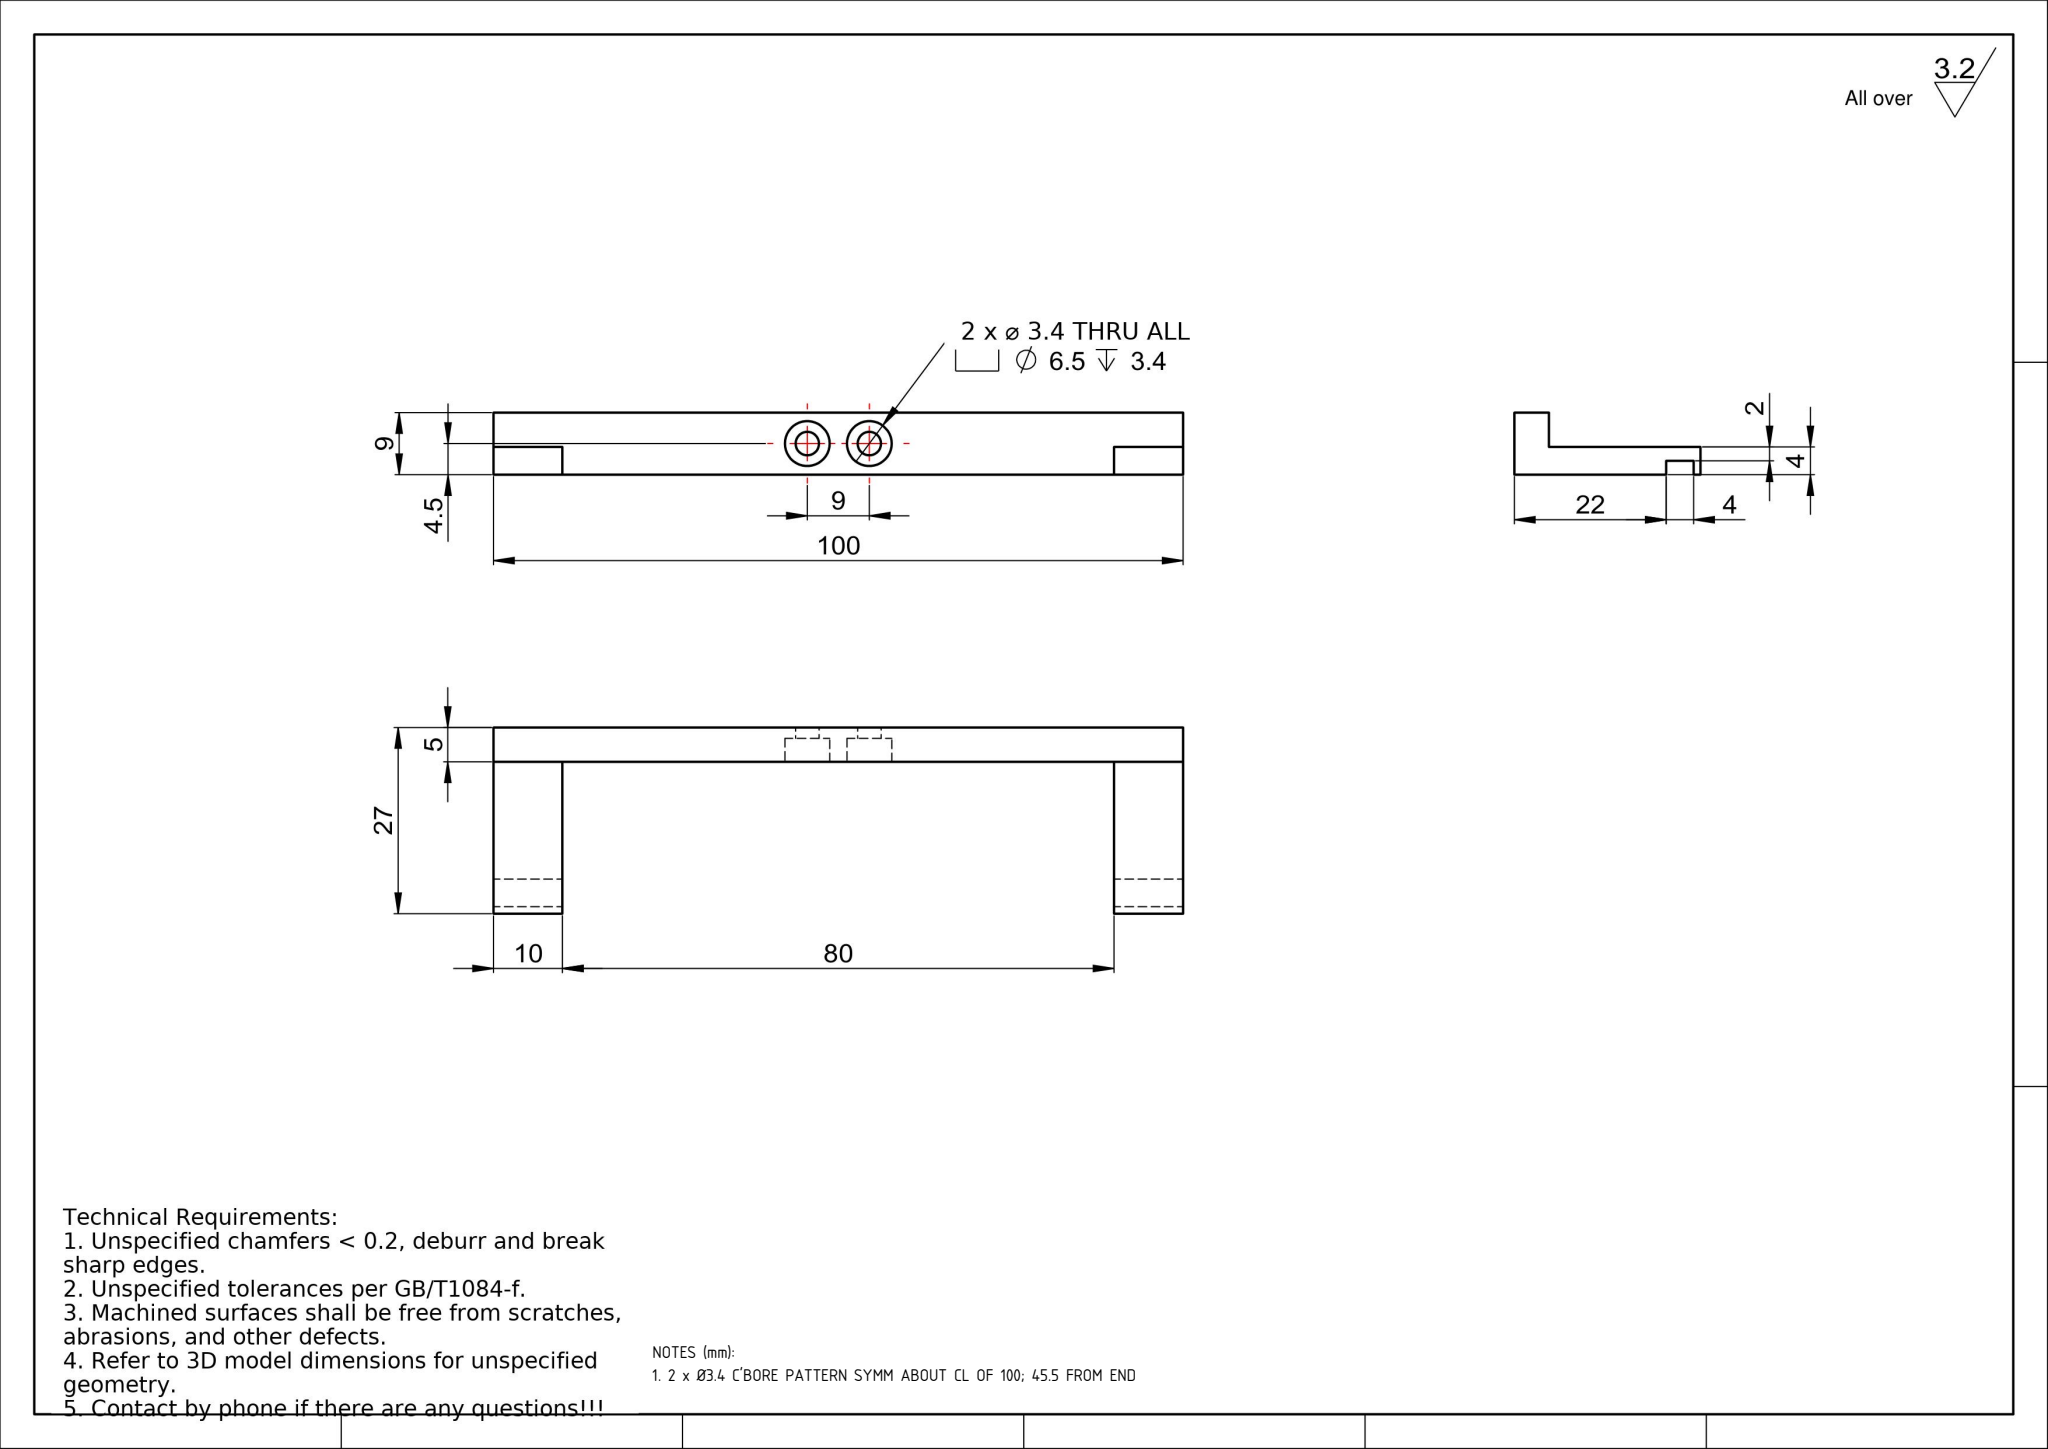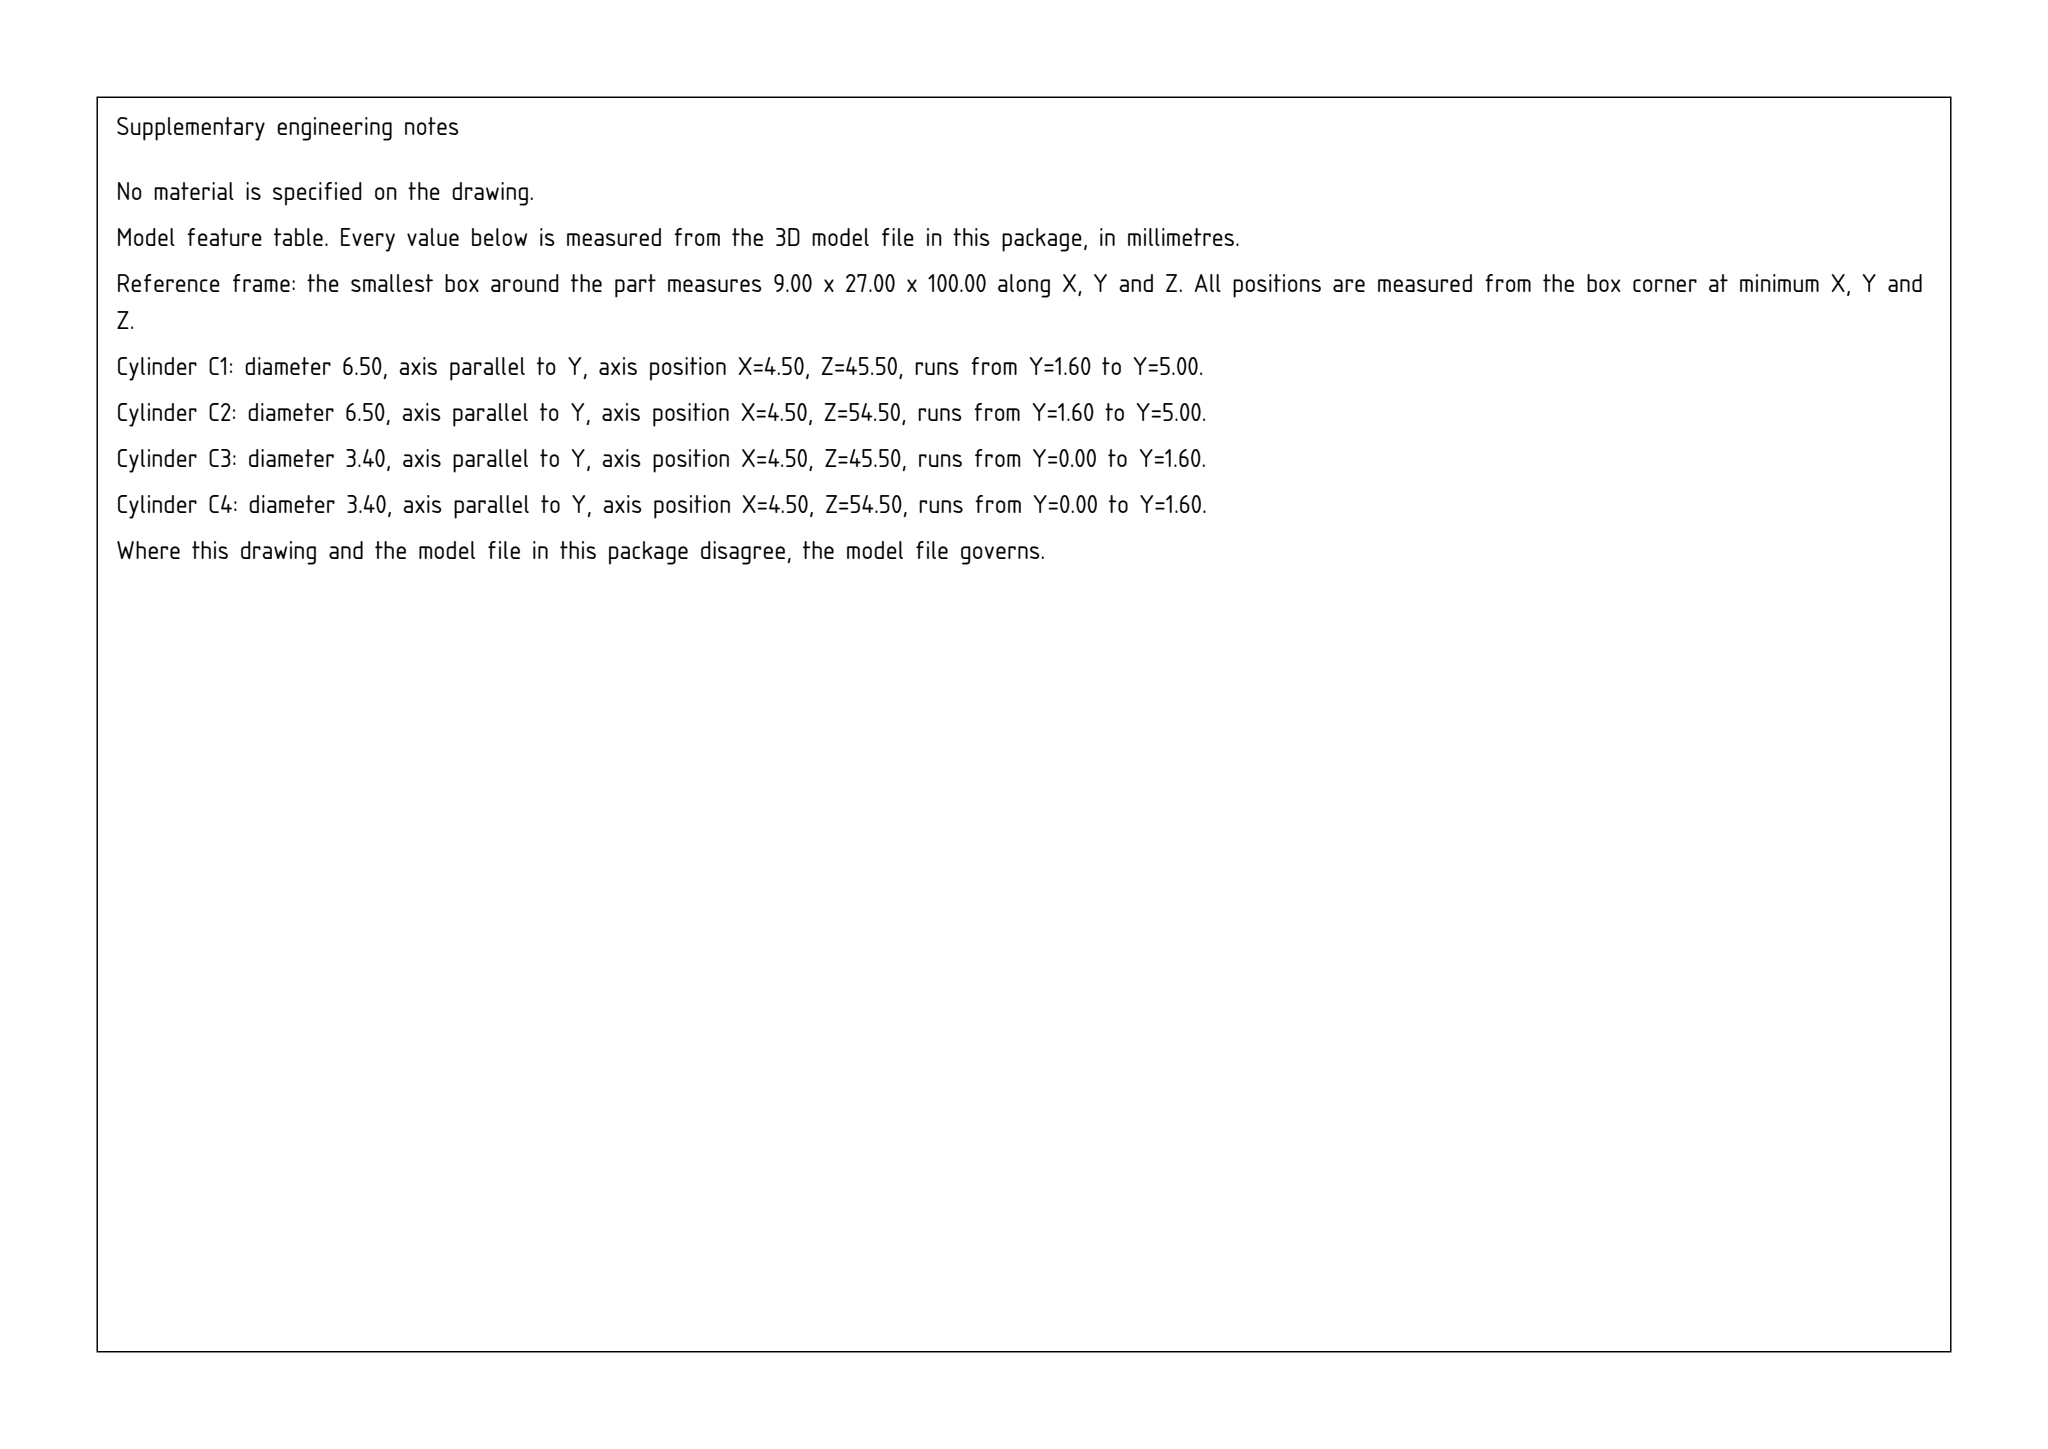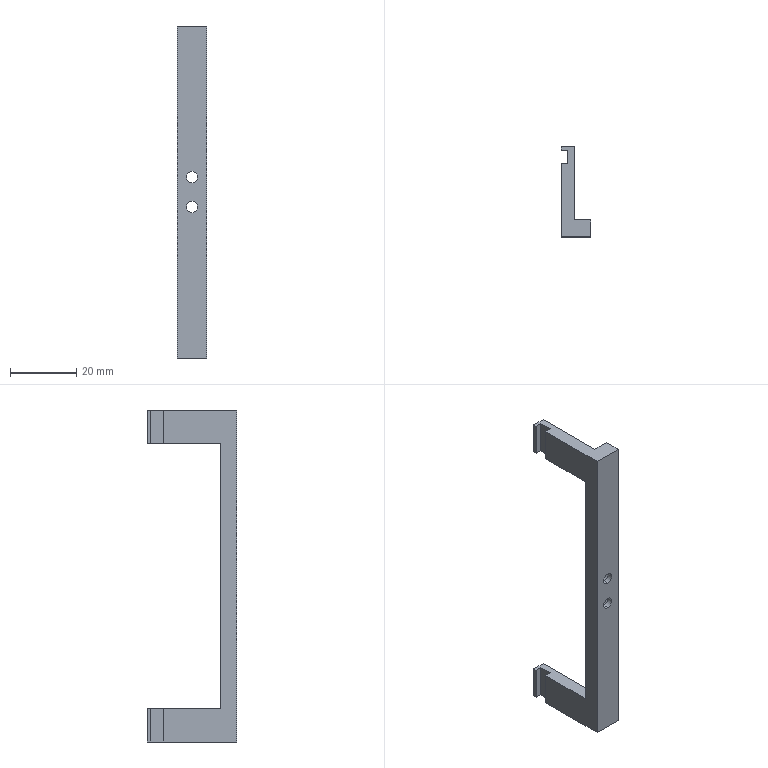Part | SolidWorks | mm | 1 solid | 30 faces | box 9 x 27 x 100 mm | volume 5845 mm3 | plane 22 | cylinder 8 | commonest cylinder face diameters 6.5 x4 3.4 x4
Drawing notes:
2 x Ø3.4 C'BORE PATTERN SYMM ABOUT CL OF 100; 45.5 FROM END | from the solid: Ø3.4/Ø6.5 axes at z=45.5 and 54.5 of 100 length (symmetric about z=50), 9 apart
build123d program:
from build123d import *

# Parameters (mm, degrees)
BOSS_EXTRUDE1_DEPTH                             = 50
SKETCH2_W                                       = 80
SKETCH2_H                                       = 22
CUT_EXTRUDE1_DEPTH                              = 58.044
SKETCH3_W                                       = 2
SKETCH3_H                                       = 4
CUT_EXTRUDE2_DEPTH                              = 104.971
M3_HEX_SOCKET_HEAD_CAP_SCREW_CBORE1_D           = 3.4
M3_HEX_SOCKET_HEAD_CAP_SCREW_CBORE1_CBORE_D     = 6.5
M3_HEX_SOCKET_HEAD_CAP_SCREW_CBORE1_CBORE_DEPTH = 3.4


with BuildPart() as part:
    # Sketch1 → Boss-Extrude1 (new, symmetric)
    with BuildSketch(Plane.XY):
        Polygon((0, 0), (0, 27), (4, 27), (4, 5), (9, 5), (9, 0), align=None)
    extrude(amount=BOSS_EXTRUDE1_DEPTH, both=True)

    # Sketch2 → Cut-Extrude1 (cut, through all)
    with BuildSketch(Plane(origin=(4, 0, 0), x_dir=(0, 0, -1), z_dir=(1, 0, 0))):
        with Locations((0, 16)):
            Rectangle(SKETCH2_W, SKETCH2_H)
    extrude(amount=-CUT_EXTRUDE1_DEPTH, mode=Mode.SUBTRACT)

    # Sketch3 → Cut-Extrude2 (cut, through all)
    with BuildSketch(Plane.XY.offset(50)):
        with Locations((1, 24)):
            Rectangle(SKETCH3_W, SKETCH3_H)
    extrude(amount=-CUT_EXTRUDE2_DEPTH, mode=Mode.SUBTRACT)

    # M3 Hex Socket Head Cap Screw CBORE1 (through all)
    with Locations(Plane(origin=(0, 5, 0), x_dir=(1, 0, 0), z_dir=(0, 1, 0))):
        with Locations((4.5, 4.5), (4.5, -4.5)):
            CounterBoreHole(M3_HEX_SOCKET_HEAD_CAP_SCREW_CBORE1_D / 2, M3_HEX_SOCKET_HEAD_CAP_SCREW_CBORE1_CBORE_D / 2, M3_HEX_SOCKET_HEAD_CAP_SCREW_CBORE1_CBORE_DEPTH)


solid = part.part
STEP:
#1=CARTESIAN_POINT('',(4.5,1.6,-7.75));
#2=VERTEX_POINT('',#1);
#3=CARTESIAN_POINT('',(4.5,1.6,-1.25));
#4=VERTEX_POINT('',#3);
#5=CARTESIAN_POINT('',(4.5,1.6,-4.5));
#6=DIRECTION('',(0.,1.,0.));
#7=DIRECTION('',(0.,0.,1.));
#8=AXIS2_PLACEMENT_3D('',#5,#6,#7);
#9=CIRCLE('',#8,3.25);
#10=EDGE_CURVE('',#2,#4,#9,.T.);
#11=ORIENTED_EDGE('',*,*,#10,.F.);
#12=CARTESIAN_POINT('',(4.5,5.,-7.75));
#13=VERTEX_POINT('',#12);
#14=CARTESIAN_POINT('',(4.5,5.,-7.75));
#15=DIRECTION('',(0.,1.,0.));
#16=VECTOR('',#15,1000.);
#17=LINE('',#14,#16);
#18=EDGE_CURVE('',#2,#13,#17,.T.);
#19=ORIENTED_EDGE('',*,*,#18,.T.);
#20=CARTESIAN_POINT('',(4.5,5.,-1.25));
#21=VERTEX_POINT('',#20);
#22=CARTESIAN_POINT('',(4.5,5.,-4.5));
#23=DIRECTION('',(0.,1.,0.));
#24=DIRECTION('',(0.,0.,1.));
#25=AXIS2_PLACEMENT_3D('',#22,#23,#24);
#26=CIRCLE('',#25,3.25);
#27=EDGE_CURVE('',#13,#21,#26,.T.);
#28=ORIENTED_EDGE('',*,*,#27,.T.);
#29=CARTESIAN_POINT('',(4.5,5.,-1.25));
#30=DIRECTION('',(0.,1.,0.));
#31=VECTOR('',#30,1000.);
#32=LINE('',#29,#31);
#33=EDGE_CURVE('',#4,#21,#32,.T.);
#34=ORIENTED_EDGE('',*,*,#33,.F.);
#35=EDGE_LOOP('',(#11,#19,#28,#34));
#36=FACE_OUTER_BOUND('',#35,.T.);
#37=CARTESIAN_POINT('',(4.5,5.,-4.5));
#38=DIRECTION('',(0.,1.,0.));
#39=DIRECTION('',(0.,0.,1.));
#40=AXIS2_PLACEMENT_3D('',#37,#38,#39);
#41=CYLINDRICAL_SURFACE('',#40,3.25);
#42=ADVANCED_FACE('',(#36),#41,.F.);
#43=CARTESIAN_POINT('',(4.5,-0.,-6.2));
#44=VERTEX_POINT('',#43);
#45=CARTESIAN_POINT('',(4.5,-0.,-2.8));
#46=VERTEX_POINT('',#45);
#47=CARTESIAN_POINT('',(4.5,-0.,-4.5));
#48=DIRECTION('',(0.,1.,0.));
#49=DIRECTION('',(0.,0.,1.));
#50=AXIS2_PLACEMENT_3D('',#47,#48,#49);
#51=CIRCLE('',#50,1.7);
#52=EDGE_CURVE('',#44,#46,#51,.T.);
#53=ORIENTED_EDGE('',*,*,#52,.F.);
#54=CARTESIAN_POINT('',(4.5,1.6,-6.2));
#55=VERTEX_POINT('',#54);
#56=CARTESIAN_POINT('',(4.5,5.,-6.2));
#57=DIRECTION('',(0.,1.,0.));
#58=VECTOR('',#57,1000.);
#59=LINE('',#56,#58);
#60=EDGE_CURVE('',#44,#55,#59,.T.);
#61=ORIENTED_EDGE('',*,*,#60,.T.);
#62=CARTESIAN_POINT('',(4.5,1.6,-2.8));
#63=VERTEX_POINT('',#62);
#64=CARTESIAN_POINT('',(4.5,1.6,-4.5));
#65=DIRECTION('',(0.,1.,0.));
#66=DIRECTION('',(0.,0.,1.));
#67=AXIS2_PLACEMENT_3D('',#64,#65,#66);
#68=CIRCLE('',#67,1.7);
#69=EDGE_CURVE('',#55,#63,#68,.T.);
#70=ORIENTED_EDGE('',*,*,#69,.T.);
#71=CARTESIAN_POINT('',(4.5,5.,-2.8));
#72=DIRECTION('',(0.,1.,0.));
#73=VECTOR('',#72,1000.);
#74=LINE('',#71,#73);
#75=EDGE_CURVE('',#46,#63,#74,.T.);
#76=ORIENTED_EDGE('',*,*,#75,.F.);
#77=EDGE_LOOP('',(#53,#61,#70,#76));
#78=FACE_OUTER_BOUND('',#77,.T.);
#79=CARTESIAN_POINT('',(4.5,5.,-4.5));
#80=DIRECTION('',(0.,1.,0.));
#81=DIRECTION('',(0.,0.,1.));
#82=AXIS2_PLACEMENT_3D('',#79,#80,#81);
#83=CYLINDRICAL_SURFACE('',#82,1.7);
#84=ADVANCED_FACE('',(#78),#83,.F.);
#85=CARTESIAN_POINT('',(4.5,1.6,1.25));
#86=VERTEX_POINT('',#85);
#87=CARTESIAN_POINT('',(4.5,1.6,7.75));
#88=VERTEX_POINT('',#87);
#89=CARTESIAN_POINT('',(4.5,1.6,4.5));
#90=DIRECTION('',(0.,1.,0.));
#91=DIRECTION('',(0.,0.,1.));
#92=AXIS2_PLACEMENT_3D('',#89,#90,#91);
#93=CIRCLE('',#92,3.25);
#94=EDGE_CURVE('',#86,#88,#93,.T.);
#95=ORIENTED_EDGE('',*,*,#94,.F.);
#96=CARTESIAN_POINT('',(4.5,5.,1.25));
#97=VERTEX_POINT('',#96);
#98=CARTESIAN_POINT('',(4.5,5.,1.25));
#99=DIRECTION('',(0.,1.,0.));
#100=VECTOR('',#99,1000.);
#101=LINE('',#98,#100);
#102=EDGE_CURVE('',#86,#97,#101,.T.);
#103=ORIENTED_EDGE('',*,*,#102,.T.);
#104=CARTESIAN_POINT('',(4.5,5.,7.75));
#105=VERTEX_POINT('',#104);
#106=CARTESIAN_POINT('',(4.5,5.,4.5));
#107=DIRECTION('',(0.,1.,0.));
#108=DIRECTION('',(0.,0.,1.));
#109=AXIS2_PLACEMENT_3D('',#106,#107,#108);
#110=CIRCLE('',#109,3.25);
#111=EDGE_CURVE('',#97,#105,#110,.T.);
#112=ORIENTED_EDGE('',*,*,#111,.T.);
#113=CARTESIAN_POINT('',(4.5,5.,7.75));
#114=DIRECTION('',(0.,1.,0.));
#115=VECTOR('',#114,1000.);
#116=LINE('',#113,#115);
#117=EDGE_CURVE('',#88,#105,#116,.T.);
#118=ORIENTED_EDGE('',*,*,#117,.F.);
#119=EDGE_LOOP('',(#95,#103,#112,#118));
#120=FACE_OUTER_BOUND('',#119,.T.);
#121=CARTESIAN_POINT('',(4.5,5.,4.5));
#122=DIRECTION('',(0.,1.,0.));
#123=DIRECTION('',(0.,0.,1.));
#124=AXIS2_PLACEMENT_3D('',#121,#122,#123);
#125=CYLINDRICAL_SURFACE('',#124,3.25);
#126=ADVANCED_FACE('',(#120),#125,.F.);
#127=CARTESIAN_POINT('',(4.5,-0.,2.8));
#128=VERTEX_POINT('',#127);
#129=CARTESIAN_POINT('',(4.5,-0.,6.2));
#130=VERTEX_POINT('',#129);
#131=CARTESIAN_POINT('',(4.5,-0.,4.5));
#132=DIRECTION('',(0.,1.,0.));
#133=DIRECTION('',(0.,0.,1.));
#134=AXIS2_PLACEMENT_3D('',#131,#132,#133);
#135=CIRCLE('',#134,1.7);
#136=EDGE_CURVE('',#128,#130,#135,.T.);
#137=ORIENTED_EDGE('',*,*,#136,.F.);
#138=CARTESIAN_POINT('',(4.5,1.6,2.8));
#139=VERTEX_POINT('',#138);
#140=CARTESIAN_POINT('',(4.5,5.,2.8));
#141=DIRECTION('',(0.,1.,0.));
#142=VECTOR('',#141,1000.);
#143=LINE('',#140,#142);
#144=EDGE_CURVE('',#128,#139,#143,.T.);
#145=ORIENTED_EDGE('',*,*,#144,.T.);
#146=CARTESIAN_POINT('',(4.5,1.6,6.2));
#147=VERTEX_POINT('',#146);
#148=CARTESIAN_POINT('',(4.5,1.6,4.5));
#149=DIRECTION('',(0.,1.,0.));
#150=DIRECTION('',(0.,0.,1.));
#151=AXIS2_PLACEMENT_3D('',#148,#149,#150);
#152=CIRCLE('',#151,1.7);
#153=EDGE_CURVE('',#139,#147,#152,.T.);
#154=ORIENTED_EDGE('',*,*,#153,.T.);
#155=CARTESIAN_POINT('',(4.5,5.,6.2));
#156=DIRECTION('',(0.,1.,0.));
#157=VECTOR('',#156,1000.);
#158=LINE('',#155,#157);
#159=EDGE_CURVE('',#130,#147,#158,.T.);
#160=ORIENTED_EDGE('',*,*,#159,.F.);
#161=EDGE_LOOP('',(#137,#145,#154,#160));
#162=FACE_OUTER_BOUND('',#161,.T.);
#163=CARTESIAN_POINT('',(4.5,5.,4.5));
#164=DIRECTION('',(0.,1.,0.));
#165=DIRECTION('',(0.,0.,1.));
#166=AXIS2_PLACEMENT_3D('',#163,#164,#165);
#167=CYLINDRICAL_SURFACE('',#166,1.7);
#168=ADVANCED_FACE('',(#162),#167,.F.);
#169=CARTESIAN_POINT('',(-0.,27.,40.));
#170=VERTEX_POINT('',#169);
#171=CARTESIAN_POINT('',(0.,26.,40.));
#172=VERTEX_POINT('',#171);
#173=CARTESIAN_POINT('',(-0.,27.,40.));
#174=DIRECTION('',(0.,-1.,0.));
#175=VECTOR('',#174,1000.);
#176=LINE('',#173,#175);
#177=EDGE_CURVE('',#170,#172,#176,.T.);
#178=ORIENTED_EDGE('',*,*,#177,.T.);
#179=CARTESIAN_POINT('',(0.,26.,50.));
#180=VERTEX_POINT('',#179);
#181=CARTESIAN_POINT('',(0.,26.,-50.));
#182=DIRECTION('',(0.,0.,1.));
#183=VECTOR('',#182,1000.);
#184=LINE('',#181,#183);
#185=EDGE_CURVE('',#172,#180,#184,.T.);
#186=ORIENTED_EDGE('',*,*,#185,.T.);
#187=CARTESIAN_POINT('',(0.,27.,50.));
#188=VERTEX_POINT('',#187);
#189=CARTESIAN_POINT('',(0.,0.,50.));
#190=DIRECTION('',(0.,-1.,0.));
#191=VECTOR('',#190,1000.);
#192=LINE('',#189,#191);
#193=EDGE_CURVE('',#188,#180,#192,.T.);
#194=ORIENTED_EDGE('',*,*,#193,.F.);
#195=CARTESIAN_POINT('',(0.,27.,50.));
#196=DIRECTION('',(0.,0.,-1.));
#197=VECTOR('',#196,1000.);
#198=LINE('',#195,#197);
#199=EDGE_CURVE('',#188,#170,#198,.T.);
#200=ORIENTED_EDGE('',*,*,#199,.T.);
#201=EDGE_LOOP('',(#178,#186,#194,#200));
#202=FACE_OUTER_BOUND('',#201,.T.);
#203=CARTESIAN_POINT('',(0.,0.,50.));
#204=DIRECTION('',(1.,0.,0.));
#205=DIRECTION('',(0.,0.,-1.));
#206=AXIS2_PLACEMENT_3D('',#203,#204,#205);
#207=PLANE('',#206);
#208=ADVANCED_FACE('',(#202),#207,.F.);
#209=CARTESIAN_POINT('',(0.,27.,-50.));
#210=VERTEX_POINT('',#209);
#211=CARTESIAN_POINT('',(0.,26.,-50.));
#212=VERTEX_POINT('',#211);
#213=CARTESIAN_POINT('',(0.,0.,-50.));
#214=DIRECTION('',(0.,-1.,0.));
#215=VECTOR('',#214,1000.);
#216=LINE('',#213,#215);
#217=EDGE_CURVE('',#210,#212,#216,.T.);
#218=ORIENTED_EDGE('',*,*,#217,.T.);
#219=CARTESIAN_POINT('',(0.,26.,-40.));
#220=VERTEX_POINT('',#219);
#221=CARTESIAN_POINT('',(0.,26.,-50.));
#222=DIRECTION('',(0.,0.,1.));
#223=VECTOR('',#222,1000.);
#224=LINE('',#221,#223);
#225=EDGE_CURVE('',#212,#220,#224,.T.);
#226=ORIENTED_EDGE('',*,*,#225,.T.);
#227=CARTESIAN_POINT('',(-0.,27.,-40.));
#228=VERTEX_POINT('',#227);
#229=CARTESIAN_POINT('',(-0.,27.,-40.));
#230=DIRECTION('',(-0.,1.,0.));
#231=VECTOR('',#230,1000.);
#232=LINE('',#229,#231);
#233=EDGE_CURVE('',#220,#228,#232,.T.);
#234=ORIENTED_EDGE('',*,*,#233,.T.);
#235=CARTESIAN_POINT('',(0.,27.,50.));
#236=DIRECTION('',(0.,0.,-1.));
#237=VECTOR('',#236,1000.);
#238=LINE('',#235,#237);
#239=EDGE_CURVE('',#228,#210,#238,.T.);
#240=ORIENTED_EDGE('',*,*,#239,.T.);
#241=EDGE_LOOP('',(#218,#226,#234,#240));
#242=FACE_OUTER_BOUND('',#241,.T.);
#243=CARTESIAN_POINT('',(0.,0.,50.));
#244=DIRECTION('',(1.,0.,0.));
#245=DIRECTION('',(0.,0.,-1.));
#246=AXIS2_PLACEMENT_3D('',#243,#244,#245);
#247=PLANE('',#246);
#248=ADVANCED_FACE('',(#242),#247,.F.);
#249=CARTESIAN_POINT('',(4.,5.,50.));
#250=VERTEX_POINT('',#249);
#251=CARTESIAN_POINT('',(4.,5.,40.));
#252=VERTEX_POINT('',#251);
#253=CARTESIAN_POINT('',(4.,5.,50.));
#254=DIRECTION('',(0.,0.,-1.));
#255=VECTOR('',#254,1000.);
#256=LINE('',#253,#255);
#257=EDGE_CURVE('',#250,#252,#256,.T.);
#258=ORIENTED_EDGE('',*,*,#257,.T.);
#259=CARTESIAN_POINT('',(4.,27.,40.));
#260=VERTEX_POINT('',#259);
#261=CARTESIAN_POINT('',(4.,27.,40.));
#262=DIRECTION('',(0.,-1.,0.));
#263=VECTOR('',#262,1000.);
#264=LINE('',#261,#263);
#265=EDGE_CURVE('',#260,#252,#264,.T.);
#266=ORIENTED_EDGE('',*,*,#265,.F.);
#267=CARTESIAN_POINT('',(4.,27.,50.));
#268=VERTEX_POINT('',#267);
#269=CARTESIAN_POINT('',(4.,27.,50.));
#270=DIRECTION('',(0.,0.,-1.));
#271=VECTOR('',#270,1000.);
#272=LINE('',#269,#271);
#273=EDGE_CURVE('',#268,#260,#272,.T.);
#274=ORIENTED_EDGE('',*,*,#273,.F.);
#275=CARTESIAN_POINT('',(4.,27.,50.));
#276=DIRECTION('',(-0.,1.,0.));
#277=VECTOR('',#276,1000.);
#278=LINE('',#275,#277);
#279=EDGE_CURVE('',#250,#268,#278,.T.);
#280=ORIENTED_EDGE('',*,*,#279,.F.);
#281=EDGE_LOOP('',(#258,#266,#274,#280));
#282=FACE_OUTER_BOUND('',#281,.T.);
#283=CARTESIAN_POINT('',(4.,27.,50.));
#284=DIRECTION('',(-1.,-0.,0.));
#285=DIRECTION('',(0.,-1.,0.));
#286=AXIS2_PLACEMENT_3D('',#283,#284,#285);
#287=PLANE('',#286);
#288=ADVANCED_FACE('',(#282),#287,.F.);
#289=ORIENTED_EDGE('',*,*,#273,.T.);
#290=CARTESIAN_POINT('',(-0.,27.,40.));
#291=DIRECTION('',(1.,0.,0.));
#292=VECTOR('',#291,1000.);
#293=LINE('',#290,#292);
#294=EDGE_CURVE('',#170,#260,#293,.T.);
#295=ORIENTED_EDGE('',*,*,#294,.F.);
#296=ORIENTED_EDGE('',*,*,#199,.F.);
#297=CARTESIAN_POINT('',(0.,27.,50.));
#298=DIRECTION('',(-1.,0.,0.));
#299=VECTOR('',#298,1000.);
#300=LINE('',#297,#299);
#301=EDGE_CURVE('',#268,#188,#300,.T.);
#302=ORIENTED_EDGE('',*,*,#301,.F.);
#303=EDGE_LOOP('',(#289,#295,#296,#302));
#304=FACE_OUTER_BOUND('',#303,.T.);
#305=CARTESIAN_POINT('',(0.,27.,50.));
#306=DIRECTION('',(0.,-1.,0.));
#307=DIRECTION('',(0.,0.,-1.));
#308=AXIS2_PLACEMENT_3D('',#305,#306,#307);
#309=PLANE('',#308);
#310=ADVANCED_FACE('',(#304),#309,.F.);
#311=CARTESIAN_POINT('',(4.5,-0.,-4.5));
#312=DIRECTION('',(0.,1.,0.));
#313=DIRECTION('',(0.,0.,1.));
#314=AXIS2_PLACEMENT_3D('',#311,#312,#313);
#315=CIRCLE('',#314,1.7);
#316=EDGE_CURVE('',#46,#44,#315,.T.);
#317=ORIENTED_EDGE('',*,*,#316,.T.);
#318=ORIENTED_EDGE('',*,*,#52,.T.);
#319=EDGE_LOOP('',(#317,#318));
#320=FACE_BOUND('',#319,.T.);
#321=CARTESIAN_POINT('',(4.5,-0.,4.5));
#322=DIRECTION('',(0.,1.,0.));
#323=DIRECTION('',(0.,0.,1.));
#324=AXIS2_PLACEMENT_3D('',#321,#322,#323);
#325=CIRCLE('',#324,1.7);
#326=EDGE_CURVE('',#130,#128,#325,.T.);
#327=ORIENTED_EDGE('',*,*,#326,.T.);
#328=ORIENTED_EDGE('',*,*,#136,.T.);
#329=EDGE_LOOP('',(#327,#328));
#330=FACE_BOUND('',#329,.T.);
#331=CARTESIAN_POINT('',(0.,0.,-50.));
#332=VERTEX_POINT('',#331);
#333=CARTESIAN_POINT('',(9.,-0.,-50.));
#334=VERTEX_POINT('',#333);
#335=CARTESIAN_POINT('',(9.,-0.,-50.));
#336=DIRECTION('',(1.,-0.,0.));
#337=VECTOR('',#336,1000.);
#338=LINE('',#335,#337);
#339=EDGE_CURVE('',#332,#334,#338,.T.);
#340=ORIENTED_EDGE('',*,*,#339,.T.);
#341=CARTESIAN_POINT('',(9.,-0.,50.));
#342=VERTEX_POINT('',#341);
#343=CARTESIAN_POINT('',(9.,-0.,50.));
#344=DIRECTION('',(0.,0.,-1.));
#345=VECTOR('',#344,1000.);
#346=LINE('',#343,#345);
#347=EDGE_CURVE('',#342,#334,#346,.T.);
#348=ORIENTED_EDGE('',*,*,#347,.F.);
#349=CARTESIAN_POINT('',(0.,0.,50.));
#350=VERTEX_POINT('',#349);
#351=CARTESIAN_POINT('',(9.,-0.,50.));
#352=DIRECTION('',(1.,-0.,0.));
#353=VECTOR('',#352,1000.);
#354=LINE('',#351,#353);
#355=EDGE_CURVE('',#350,#342,#354,.T.);
#356=ORIENTED_EDGE('',*,*,#355,.F.);
#357=CARTESIAN_POINT('',(0.,0.,50.));
#358=DIRECTION('',(0.,0.,-1.));
#359=VECTOR('',#358,1000.);
#360=LINE('',#357,#359);
#361=EDGE_CURVE('',#350,#332,#360,.T.);
#362=ORIENTED_EDGE('',*,*,#361,.T.);
#363=EDGE_LOOP('',(#340,#348,#356,#362));
#364=FACE_OUTER_BOUND('',#363,.T.);
#365=CARTESIAN_POINT('',(9.,-0.,50.));
#366=DIRECTION('',(0.,1.,0.));
#367=DIRECTION('',(-1.,0.,0.));
#368=AXIS2_PLACEMENT_3D('',#365,#366,#367);
#369=PLANE('',#368);
#370=ADVANCED_FACE('',(#320,#330,#364),#369,.F.);
#371=CARTESIAN_POINT('',(9.,5.,-50.));
#372=VERTEX_POINT('',#371);
#373=CARTESIAN_POINT('',(9.,5.,-50.));
#374=DIRECTION('',(-0.,1.,0.));
#375=VECTOR('',#374,1000.);
#376=LINE('',#373,#375);
#377=EDGE_CURVE('',#334,#372,#376,.T.);
#378=ORIENTED_EDGE('',*,*,#377,.T.);
#379=CARTESIAN_POINT('',(9.,5.,50.));
#380=VERTEX_POINT('',#379);
#381=CARTESIAN_POINT('',(9.,5.,50.));
#382=DIRECTION('',(0.,0.,-1.));
#383=VECTOR('',#382,1000.);
#384=LINE('',#381,#383);
#385=EDGE_CURVE('',#380,#372,#384,.T.);
#386=ORIENTED_EDGE('',*,*,#385,.F.);
#387=CARTESIAN_POINT('',(9.,5.,50.));
#388=DIRECTION('',(-0.,1.,0.));
#389=VECTOR('',#388,1000.);
#390=LINE('',#387,#389);
#391=EDGE_CURVE('',#342,#380,#390,.T.);
#392=ORIENTED_EDGE('',*,*,#391,.F.);
#393=ORIENTED_EDGE('',*,*,#347,.T.);
#394=EDGE_LOOP('',(#378,#386,#392,#393));
#395=FACE_OUTER_BOUND('',#394,.T.);
#396=CARTESIAN_POINT('',(9.,5.,50.));
#397=DIRECTION('',(-1.,-0.,0.));
#398=DIRECTION('',(0.,-1.,0.));
#399=AXIS2_PLACEMENT_3D('',#396,#397,#398);
#400=PLANE('',#399);
#401=ADVANCED_FACE('',(#395),#400,.F.);
#402=CARTESIAN_POINT('',(4.5,5.,-4.5));
#403=DIRECTION('',(0.,1.,0.));
#404=DIRECTION('',(0.,0.,1.));
#405=AXIS2_PLACEMENT_3D('',#402,#403,#404);
#406=CIRCLE('',#405,3.25);
#407=EDGE_CURVE('',#21,#13,#406,.T.);
#408=ORIENTED_EDGE('',*,*,#407,.F.);
#409=ORIENTED_EDGE('',*,*,#27,.F.);
#410=EDGE_LOOP('',(#408,#409));
#411=FACE_BOUND('',#410,.T.);
#412=CARTESIAN_POINT('',(4.5,5.,4.5));
#413=DIRECTION('',(0.,1.,0.));
#414=DIRECTION('',(0.,0.,1.));
#415=AXIS2_PLACEMENT_3D('',#412,#413,#414);
#416=CIRCLE('',#415,3.25);
#417=EDGE_CURVE('',#105,#97,#416,.T.);
#418=ORIENTED_EDGE('',*,*,#417,.F.);
#419=ORIENTED_EDGE('',*,*,#111,.F.);
#420=EDGE_LOOP('',(#418,#419));
#421=FACE_BOUND('',#420,.T.);
#422=CARTESIAN_POINT('',(4.,5.,-50.));
#423=VERTEX_POINT('',#422);
#424=CARTESIAN_POINT('',(4.,5.,-50.));
#425=DIRECTION('',(-1.,0.,0.));
#426=VECTOR('',#425,1000.);
#427=LINE('',#424,#426);
#428=EDGE_CURVE('',#372,#423,#427,.T.);
#429=ORIENTED_EDGE('',*,*,#428,.T.);
#430=CARTESIAN_POINT('',(4.,5.,-40.));
#431=VERTEX_POINT('',#430);
#432=CARTESIAN_POINT('',(4.,5.,50.));
#433=DIRECTION('',(0.,0.,-1.));
#434=VECTOR('',#433,1000.);
#435=LINE('',#432,#434);
#436=EDGE_CURVE('',#431,#423,#435,.T.);
#437=ORIENTED_EDGE('',*,*,#436,.F.);
#438=CARTESIAN_POINT('',(0.,5.,-40.));
#439=VERTEX_POINT('',#438);
#440=CARTESIAN_POINT('',(-0.,5.,-40.));
#441=DIRECTION('',(1.,0.,0.));
#442=VECTOR('',#441,1000.);
#443=LINE('',#440,#442);
#444=EDGE_CURVE('',#439,#431,#443,.T.);
#445=ORIENTED_EDGE('',*,*,#444,.F.);
#446=CARTESIAN_POINT('',(-0.,5.,40.));
#447=VERTEX_POINT('',#446);
#448=CARTESIAN_POINT('',(-0.,5.,40.));
#449=DIRECTION('',(0.,0.,-1.));
#450=VECTOR('',#449,1000.);
#451=LINE('',#448,#450);
#452=EDGE_CURVE('',#447,#439,#451,.T.);
#453=ORIENTED_EDGE('',*,*,#452,.F.);
#454=CARTESIAN_POINT('',(-0.,5.,40.));
#455=DIRECTION('',(1.,0.,0.));
#456=VECTOR('',#455,1000.);
#457=LINE('',#454,#456);
#458=EDGE_CURVE('',#447,#252,#457,.T.);
#459=ORIENTED_EDGE('',*,*,#458,.T.);
#460=ORIENTED_EDGE('',*,*,#257,.F.);
#461=CARTESIAN_POINT('',(4.,5.,50.));
#462=DIRECTION('',(-1.,0.,0.));
#463=VECTOR('',#462,1000.);
#464=LINE('',#461,#463);
#465=EDGE_CURVE('',#380,#250,#464,.T.);
#466=ORIENTED_EDGE('',*,*,#465,.F.);
#467=ORIENTED_EDGE('',*,*,#385,.T.);
#468=EDGE_LOOP('',(#429,#437,#445,#453,#459,#460,#466,#467));
#469=FACE_OUTER_BOUND('',#468,.T.);
#470=CARTESIAN_POINT('',(4.,5.,50.));
#471=DIRECTION('',(-0.,-1.,0.));
#472=DIRECTION('',(1.,-0.,0.));
#473=AXIS2_PLACEMENT_3D('',#470,#471,#472);
#474=PLANE('',#473);
#475=ADVANCED_FACE('',(#411,#421,#469),#474,.F.);
#476=CARTESIAN_POINT('',(4.,27.,-40.));
#477=VERTEX_POINT('',#476);
#478=CARTESIAN_POINT('',(4.,27.,-50.));
#479=VERTEX_POINT('',#478);
#480=CARTESIAN_POINT('',(4.,27.,50.));
#481=DIRECTION('',(0.,0.,-1.));
#482=VECTOR('',#481,1000.);
#483=LINE('',#480,#482);
#484=EDGE_CURVE('',#477,#479,#483,.T.);
#485=ORIENTED_EDGE('',*,*,#484,.F.);
#486=CARTESIAN_POINT('',(4.,27.,-40.));
#487=DIRECTION('',(-0.,1.,0.));
#488=VECTOR('',#487,1000.);
#489=LINE('',#486,#488);
#490=EDGE_CURVE('',#431,#477,#489,.T.);
#491=ORIENTED_EDGE('',*,*,#490,.F.);
#492=ORIENTED_EDGE('',*,*,#436,.T.);
#493=CARTESIAN_POINT('',(4.,27.,-50.));
#494=DIRECTION('',(-0.,1.,0.));
#495=VECTOR('',#494,1000.);
#496=LINE('',#493,#495);
#497=EDGE_CURVE('',#423,#479,#496,.T.);
#498=ORIENTED_EDGE('',*,*,#497,.T.);
#499=EDGE_LOOP('',(#485,#491,#492,#498));
#500=FACE_OUTER_BOUND('',#499,.T.);
#501=CARTESIAN_POINT('',(4.,27.,50.));
#502=DIRECTION('',(-1.,-0.,0.));
#503=DIRECTION('',(0.,-1.,0.));
#504=AXIS2_PLACEMENT_3D('',#501,#502,#503);
#505=PLANE('',#504);
#506=ADVANCED_FACE('',(#500),#505,.F.);
#507=ORIENTED_EDGE('',*,*,#239,.F.);
#508=CARTESIAN_POINT('',(-0.,27.,-40.));
#509=DIRECTION('',(1.,0.,0.));
#510=VECTOR('',#509,1000.);
#511=LINE('',#508,#510);
#512=EDGE_CURVE('',#228,#477,#511,.T.);
#513=ORIENTED_EDGE('',*,*,#512,.T.);
#514=ORIENTED_EDGE('',*,*,#484,.T.);
#515=CARTESIAN_POINT('',(0.,27.,-50.));
#516=DIRECTION('',(-1.,0.,0.));
#517=VECTOR('',#516,1000.);
#518=LINE('',#515,#517);
#519=EDGE_CURVE('',#479,#210,#518,.T.);
#520=ORIENTED_EDGE('',*,*,#519,.T.);
#521=EDGE_LOOP('',(#507,#513,#514,#520));
#522=FACE_OUTER_BOUND('',#521,.T.);
#523=CARTESIAN_POINT('',(0.,27.,50.));
#524=DIRECTION('',(0.,-1.,0.));
#525=DIRECTION('',(0.,0.,-1.));
#526=AXIS2_PLACEMENT_3D('',#523,#524,#525);
#527=PLANE('',#526);
#528=ADVANCED_FACE('',(#522),#527,.F.);
#529=CARTESIAN_POINT('',(0.,22.,50.));
#530=VERTEX_POINT('',#529);
#531=CARTESIAN_POINT('',(0.,0.,50.));
#532=DIRECTION('',(0.,-1.,0.));
#533=VECTOR('',#532,1000.);
#534=LINE('',#531,#533);
#535=EDGE_CURVE('',#530,#350,#534,.T.);
#536=ORIENTED_EDGE('',*,*,#535,.F.);
#537=CARTESIAN_POINT('',(0.,22.,40.));
#538=VERTEX_POINT('',#537);
#539=CARTESIAN_POINT('',(0.,22.,-50.));
#540=DIRECTION('',(0.,0.,1.));
#541=VECTOR('',#540,1000.);
#542=LINE('',#539,#541);
#543=EDGE_CURVE('',#538,#530,#542,.T.);
#544=ORIENTED_EDGE('',*,*,#543,.F.);
#545=CARTESIAN_POINT('',(-0.,27.,40.));
#546=DIRECTION('',(0.,-1.,0.));
#547=VECTOR('',#546,1000.);
#548=LINE('',#545,#547);
#549=EDGE_CURVE('',#538,#447,#548,.T.);
#550=ORIENTED_EDGE('',*,*,#549,.T.);
#551=ORIENTED_EDGE('',*,*,#452,.T.);
#552=CARTESIAN_POINT('',(-0.,22.,-40.));
#553=VERTEX_POINT('',#552);
#554=CARTESIAN_POINT('',(-0.,27.,-40.));
#555=DIRECTION('',(-0.,1.,0.));
#556=VECTOR('',#555,1000.);
#557=LINE('',#554,#556);
#558=EDGE_CURVE('',#439,#553,#557,.T.);
#559=ORIENTED_EDGE('',*,*,#558,.T.);
#560=CARTESIAN_POINT('',(0.,22.,-50.));
#561=VERTEX_POINT('',#560);
#562=CARTESIAN_POINT('',(0.,22.,-50.));
#563=DIRECTION('',(0.,0.,1.));
#564=VECTOR('',#563,1000.);
#565=LINE('',#562,#564);
#566=EDGE_CURVE('',#561,#553,#565,.T.);
#567=ORIENTED_EDGE('',*,*,#566,.F.);
#568=CARTESIAN_POINT('',(0.,0.,-50.));
#569=DIRECTION('',(0.,-1.,0.));
#570=VECTOR('',#569,1000.);
#571=LINE('',#568,#570);
#572=EDGE_CURVE('',#561,#332,#571,.T.);
#573=ORIENTED_EDGE('',*,*,#572,.T.);
#574=ORIENTED_EDGE('',*,*,#361,.F.);
#575=EDGE_LOOP('',(#536,#544,#550,#551,#559,#567,#573,#574));
#576=FACE_OUTER_BOUND('',#575,.T.);
#577=CARTESIAN_POINT('',(0.,0.,50.));
#578=DIRECTION('',(1.,0.,0.));
#579=DIRECTION('',(0.,0.,-1.));
#580=AXIS2_PLACEMENT_3D('',#577,#578,#579);
#581=PLANE('',#580);
#582=ADVANCED_FACE('',(#576),#581,.F.);
#583=ORIENTED_EDGE('',*,*,#193,.T.);
#584=CARTESIAN_POINT('',(2.,26.,50.));
#585=VERTEX_POINT('',#584);
#586=CARTESIAN_POINT('',(0.,26.,50.));
#587=DIRECTION('',(-1.,0.,0.));
#588=VECTOR('',#587,1000.);
#589=LINE('',#586,#588);
#590=EDGE_CURVE('',#585,#180,#589,.T.);
#591=ORIENTED_EDGE('',*,*,#590,.F.);
#592=CARTESIAN_POINT('',(2.,22.,50.));
#593=VERTEX_POINT('',#592);
#594=CARTESIAN_POINT('',(2.,26.,50.));
#595=DIRECTION('',(-0.,1.,0.));
#596=VECTOR('',#595,1000.);
#597=LINE('',#594,#596);
#598=EDGE_CURVE('',#593,#585,#597,.T.);
#599=ORIENTED_EDGE('',*,*,#598,.F.);
#600=CARTESIAN_POINT('',(0.,22.,50.));
#601=DIRECTION('',(1.,0.,0.));
#602=VECTOR('',#601,1000.);
#603=LINE('',#600,#602);
#604=EDGE_CURVE('',#530,#593,#603,.T.);
#605=ORIENTED_EDGE('',*,*,#604,.F.);
#606=ORIENTED_EDGE('',*,*,#535,.T.);
#607=ORIENTED_EDGE('',*,*,#355,.T.);
#608=ORIENTED_EDGE('',*,*,#391,.T.);
#609=ORIENTED_EDGE('',*,*,#465,.T.);
#610=ORIENTED_EDGE('',*,*,#279,.T.);
#611=ORIENTED_EDGE('',*,*,#301,.T.);
#612=EDGE_LOOP('',(#583,#591,#599,#605,#606,#607,#608,#609,#610,#611));
#613=FACE_OUTER_BOUND('',#612,.T.);
#614=CARTESIAN_POINT('',(0.,0.,50.));
#615=DIRECTION('',(0.,0.,-1.));
#616=DIRECTION('',(-1.,0.,0.));
#617=AXIS2_PLACEMENT_3D('',#614,#615,#616);
#618=PLANE('',#617);
#619=ADVANCED_FACE('',(#613),#618,.F.);
#620=CARTESIAN_POINT('',(2.,26.,-50.));
#621=VERTEX_POINT('',#620);
#622=CARTESIAN_POINT('',(0.,26.,-50.));
#623=DIRECTION('',(-1.,0.,0.));
#624=VECTOR('',#623,1000.);
#625=LINE('',#622,#624);
#626=EDGE_CURVE('',#621,#212,#625,.T.);
#627=ORIENTED_EDGE('',*,*,#626,.T.);
#628=ORIENTED_EDGE('',*,*,#217,.F.);
#629=ORIENTED_EDGE('',*,*,#519,.F.);
#630=ORIENTED_EDGE('',*,*,#497,.F.);
#631=ORIENTED_EDGE('',*,*,#428,.F.);
#632=ORIENTED_EDGE('',*,*,#377,.F.);
#633=ORIENTED_EDGE('',*,*,#339,.F.);
#634=ORIENTED_EDGE('',*,*,#572,.F.);
#635=CARTESIAN_POINT('',(2.,22.,-50.));
#636=VERTEX_POINT('',#635);
#637=CARTESIAN_POINT('',(0.,22.,-50.));
#638=DIRECTION('',(1.,0.,0.));
#639=VECTOR('',#638,1000.);
#640=LINE('',#637,#639);
#641=EDGE_CURVE('',#561,#636,#640,.T.);
#642=ORIENTED_EDGE('',*,*,#641,.T.);
#643=CARTESIAN_POINT('',(2.,26.,-50.));
#644=DIRECTION('',(-0.,1.,0.));
#645=VECTOR('',#644,1000.);
#646=LINE('',#643,#645);
#647=EDGE_CURVE('',#636,#621,#646,.T.);
#648=ORIENTED_EDGE('',*,*,#647,.T.);
#649=EDGE_LOOP('',(#627,#628,#629,#630,#631,#632,#633,#634,#642,#648));
#650=FACE_OUTER_BOUND('',#649,.T.);
#651=CARTESIAN_POINT('',(0.,0.,-50.));
#652=DIRECTION('',(0.,0.,-1.));
#653=DIRECTION('',(-1.,0.,0.));
#654=AXIS2_PLACEMENT_3D('',#651,#652,#653);
#655=PLANE('',#654);
#656=ADVANCED_FACE('',(#650),#655,.T.);
#657=CARTESIAN_POINT('',(2.,22.,40.));
#658=VERTEX_POINT('',#657);
#659=CARTESIAN_POINT('',(2.,26.,40.));
#660=VERTEX_POINT('',#659);
#661=CARTESIAN_POINT('',(2.,27.,40.));
#662=DIRECTION('',(-0.,1.,-0.));
#663=VECTOR('',#662,1000.);
#664=LINE('',#661,#663);
#665=EDGE_CURVE('',#658,#660,#664,.T.);
#666=ORIENTED_EDGE('',*,*,#665,.T.);
#667=CARTESIAN_POINT('',(-0.,26.,40.));
#668=DIRECTION('',(-1.,0.,-0.));
#669=VECTOR('',#668,1000.);
#670=LINE('',#667,#669);
#671=EDGE_CURVE('',#660,#172,#670,.T.);
#672=ORIENTED_EDGE('',*,*,#671,.T.);
#673=ORIENTED_EDGE('',*,*,#177,.F.);
#674=ORIENTED_EDGE('',*,*,#294,.T.);
#675=ORIENTED_EDGE('',*,*,#265,.T.);
#676=ORIENTED_EDGE('',*,*,#458,.F.);
#677=ORIENTED_EDGE('',*,*,#549,.F.);
#678=CARTESIAN_POINT('',(-0.,22.,40.));
#679=DIRECTION('',(1.,0.,0.));
#680=VECTOR('',#679,1000.);
#681=LINE('',#678,#680);
#682=EDGE_CURVE('',#538,#658,#681,.T.);
#683=ORIENTED_EDGE('',*,*,#682,.T.);
#684=EDGE_LOOP('',(#666,#672,#673,#674,#675,#676,#677,#683));
#685=FACE_OUTER_BOUND('',#684,.T.);
#686=CARTESIAN_POINT('',(-0.,27.,40.));
#687=DIRECTION('',(-0.,0.,1.));
#688=DIRECTION('',(0.,-1.,0.));
#689=AXIS2_PLACEMENT_3D('',#686,#687,#688);
#690=PLANE('',#689);
#691=ADVANCED_FACE('',(#685),#690,.F.);
#692=ORIENTED_EDGE('',*,*,#233,.F.);
#693=CARTESIAN_POINT('',(2.,26.,-40.));
#694=VERTEX_POINT('',#693);
#695=CARTESIAN_POINT('',(-0.,26.,-40.));
#696=DIRECTION('',(1.,0.,-0.));
#697=VECTOR('',#696,1000.);
#698=LINE('',#695,#697);
#699=EDGE_CURVE('',#220,#694,#698,.T.);
#700=ORIENTED_EDGE('',*,*,#699,.T.);
#701=CARTESIAN_POINT('',(2.,22.,-40.));
#702=VERTEX_POINT('',#701);
#703=CARTESIAN_POINT('',(2.,27.,-40.));
#704=DIRECTION('',(0.,-1.,-0.));
#705=VECTOR('',#704,1000.);
#706=LINE('',#703,#705);
#707=EDGE_CURVE('',#694,#702,#706,.T.);
#708=ORIENTED_EDGE('',*,*,#707,.T.);
#709=CARTESIAN_POINT('',(-0.,22.,-40.));
#710=DIRECTION('',(-1.,0.,0.));
#711=VECTOR('',#710,1000.);
#712=LINE('',#709,#711);
#713=EDGE_CURVE('',#702,#553,#712,.T.);
#714=ORIENTED_EDGE('',*,*,#713,.T.);
#715=ORIENTED_EDGE('',*,*,#558,.F.);
#716=ORIENTED_EDGE('',*,*,#444,.T.);
#717=ORIENTED_EDGE('',*,*,#490,.T.);
#718=ORIENTED_EDGE('',*,*,#512,.F.);
#719=EDGE_LOOP('',(#692,#700,#708,#714,#715,#716,#717,#718));
#720=FACE_OUTER_BOUND('',#719,.T.);
#721=CARTESIAN_POINT('',(-0.,27.,-40.));
#722=DIRECTION('',(-0.,0.,-1.));
#723=DIRECTION('',(0.,1.,0.));
#724=AXIS2_PLACEMENT_3D('',#721,#722,#723);
#725=PLANE('',#724);
#726=ADVANCED_FACE('',(#720),#725,.F.);
#727=CARTESIAN_POINT('',(2.,22.,-50.));
#728=DIRECTION('',(0.,0.,1.));
#729=VECTOR('',#728,1000.);
#730=LINE('',#727,#729);
#731=EDGE_CURVE('',#636,#702,#730,.T.);
#732=ORIENTED_EDGE('',*,*,#731,.F.);
#733=ORIENTED_EDGE('',*,*,#641,.F.);
#734=ORIENTED_EDGE('',*,*,#566,.T.);
#735=ORIENTED_EDGE('',*,*,#713,.F.);
#736=EDGE_LOOP('',(#732,#733,#734,#735));
#737=FACE_OUTER_BOUND('',#736,.T.);
#738=CARTESIAN_POINT('',(0.,22.,-50.));
#739=DIRECTION('',(0.,-1.,0.));
#740=DIRECTION('',(0.,0.,-1.));
#741=AXIS2_PLACEMENT_3D('',#738,#739,#740);
#742=PLANE('',#741);
#743=ADVANCED_FACE('',(#737),#742,.F.);
#744=CARTESIAN_POINT('',(2.,26.,-50.));
#745=DIRECTION('',(0.,0.,1.));
#746=VECTOR('',#745,1000.);
#747=LINE('',#744,#746);
#748=EDGE_CURVE('',#621,#694,#747,.T.);
#749=ORIENTED_EDGE('',*,*,#748,.F.);
#750=ORIENTED_EDGE('',*,*,#647,.F.);
#751=ORIENTED_EDGE('',*,*,#731,.T.);
#752=ORIENTED_EDGE('',*,*,#707,.F.);
#753=EDGE_LOOP('',(#749,#750,#751,#752));
#754=FACE_OUTER_BOUND('',#753,.T.);
#755=CARTESIAN_POINT('',(2.,26.,-50.));
#756=DIRECTION('',(1.,0.,0.));
#757=DIRECTION('',(-0.,1.,0.));
#758=AXIS2_PLACEMENT_3D('',#755,#756,#757);
#759=PLANE('',#758);
#760=ADVANCED_FACE('',(#754),#759,.F.);
#761=ORIENTED_EDGE('',*,*,#225,.F.);
#762=ORIENTED_EDGE('',*,*,#626,.F.);
#763=ORIENTED_EDGE('',*,*,#748,.T.);
#764=ORIENTED_EDGE('',*,*,#699,.F.);
#765=EDGE_LOOP('',(#761,#762,#763,#764));
#766=FACE_OUTER_BOUND('',#765,.T.);
#767=CARTESIAN_POINT('',(0.,26.,-50.));
#768=DIRECTION('',(0.,1.,0.));
#769=DIRECTION('',(0.,0.,1.));
#770=AXIS2_PLACEMENT_3D('',#767,#768,#769);
#771=PLANE('',#770);
#772=ADVANCED_FACE('',(#766),#771,.F.);
#773=CARTESIAN_POINT('',(2.,26.,-50.));
#774=DIRECTION('',(0.,0.,1.));
#775=VECTOR('',#774,1000.);
#776=LINE('',#773,#775);
#777=EDGE_CURVE('',#660,#585,#776,.T.);
#778=ORIENTED_EDGE('',*,*,#777,.T.);
#779=ORIENTED_EDGE('',*,*,#590,.T.);
#780=ORIENTED_EDGE('',*,*,#185,.F.);
#781=ORIENTED_EDGE('',*,*,#671,.F.);
#782=EDGE_LOOP('',(#778,#779,#780,#781));
#783=FACE_OUTER_BOUND('',#782,.T.);
#784=CARTESIAN_POINT('',(0.,26.,-50.));
#785=DIRECTION('',(0.,1.,0.));
#786=DIRECTION('',(0.,0.,1.));
#787=AXIS2_PLACEMENT_3D('',#784,#785,#786);
#788=PLANE('',#787);
#789=ADVANCED_FACE('',(#783),#788,.F.);
#790=CARTESIAN_POINT('',(2.,22.,-50.));
#791=DIRECTION('',(0.,0.,1.));
#792=VECTOR('',#791,1000.);
#793=LINE('',#790,#792);
#794=EDGE_CURVE('',#658,#593,#793,.T.);
#795=ORIENTED_EDGE('',*,*,#794,.T.);
#796=ORIENTED_EDGE('',*,*,#598,.T.);
#797=ORIENTED_EDGE('',*,*,#777,.F.);
#798=ORIENTED_EDGE('',*,*,#665,.F.);
#799=EDGE_LOOP('',(#795,#796,#797,#798));
#800=FACE_OUTER_BOUND('',#799,.T.);
#801=CARTESIAN_POINT('',(2.,26.,-50.));
#802=DIRECTION('',(1.,0.,0.));
#803=DIRECTION('',(-0.,1.,0.));
#804=AXIS2_PLACEMENT_3D('',#801,#802,#803);
#805=PLANE('',#804);
#806=ADVANCED_FACE('',(#800),#805,.F.);
#807=ORIENTED_EDGE('',*,*,#543,.T.);
#808=ORIENTED_EDGE('',*,*,#604,.T.);
#809=ORIENTED_EDGE('',*,*,#794,.F.);
#810=ORIENTED_EDGE('',*,*,#682,.F.);
#811=EDGE_LOOP('',(#807,#808,#809,#810));
#812=FACE_OUTER_BOUND('',#811,.T.);
#813=CARTESIAN_POINT('',(0.,22.,-50.));
#814=DIRECTION('',(0.,-1.,0.));
#815=DIRECTION('',(0.,0.,-1.));
#816=AXIS2_PLACEMENT_3D('',#813,#814,#815);
#817=PLANE('',#816);
#818=ADVANCED_FACE('',(#812),#817,.F.);
#819=ORIENTED_EDGE('',*,*,#144,.F.);
#820=ORIENTED_EDGE('',*,*,#326,.F.);
#821=ORIENTED_EDGE('',*,*,#159,.T.);
#822=CARTESIAN_POINT('',(4.5,1.6,4.5));
#823=DIRECTION('',(0.,1.,0.));
#824=DIRECTION('',(0.,0.,1.));
#825=AXIS2_PLACEMENT_3D('',#822,#823,#824);
#826=CIRCLE('',#825,1.7);
#827=EDGE_CURVE('',#147,#139,#826,.T.);
#828=ORIENTED_EDGE('',*,*,#827,.T.);
#829=EDGE_LOOP('',(#819,#820,#821,#828));
#830=FACE_OUTER_BOUND('',#829,.T.);
#831=CARTESIAN_POINT('',(4.5,5.,4.5));
#832=DIRECTION('',(0.,1.,0.));
#833=DIRECTION('',(0.,0.,1.));
#834=AXIS2_PLACEMENT_3D('',#831,#832,#833);
#835=CYLINDRICAL_SURFACE('',#834,1.7);
#836=ADVANCED_FACE('',(#830),#835,.F.);
#837=ORIENTED_EDGE('',*,*,#827,.F.);
#838=ORIENTED_EDGE('',*,*,#153,.F.);
#839=EDGE_LOOP('',(#837,#838));
#840=FACE_BOUND('',#839,.T.);
#841=CARTESIAN_POINT('',(4.5,1.6,4.5));
#842=DIRECTION('',(0.,1.,0.));
#843=DIRECTION('',(0.,0.,1.));
#844=AXIS2_PLACEMENT_3D('',#841,#842,#843);
#845=CIRCLE('',#844,3.25);
#846=EDGE_CURVE('',#88,#86,#845,.T.);
#847=ORIENTED_EDGE('',*,*,#846,.T.);
#848=ORIENTED_EDGE('',*,*,#94,.T.);
#849=EDGE_LOOP('',(#847,#848));
#850=FACE_OUTER_BOUND('',#849,.T.);
#851=CARTESIAN_POINT('',(6.2,1.6,4.5));
#852=DIRECTION('',(0.,-1.,0.));
#853=DIRECTION('',(0.,0.,-1.));
#854=AXIS2_PLACEMENT_3D('',#851,#852,#853);
#855=PLANE('',#854);
#856=ADVANCED_FACE('',(#840,#850),#855,.F.);
#857=ORIENTED_EDGE('',*,*,#102,.F.);
#858=ORIENTED_EDGE('',*,*,#846,.F.);
#859=ORIENTED_EDGE('',*,*,#117,.T.);
#860=ORIENTED_EDGE('',*,*,#417,.T.);
#861=EDGE_LOOP('',(#857,#858,#859,#860));
#862=FACE_OUTER_BOUND('',#861,.T.);
#863=CARTESIAN_POINT('',(4.5,5.,4.5));
#864=DIRECTION('',(0.,1.,0.));
#865=DIRECTION('',(0.,0.,1.));
#866=AXIS2_PLACEMENT_3D('',#863,#864,#865);
#867=CYLINDRICAL_SURFACE('',#866,3.25);
#868=ADVANCED_FACE('',(#862),#867,.F.);
#869=ORIENTED_EDGE('',*,*,#60,.F.);
#870=ORIENTED_EDGE('',*,*,#316,.F.);
#871=ORIENTED_EDGE('',*,*,#75,.T.);
#872=CARTESIAN_POINT('',(4.5,1.6,-4.5));
#873=DIRECTION('',(0.,1.,0.));
#874=DIRECTION('',(0.,0.,1.));
#875=AXIS2_PLACEMENT_3D('',#872,#873,#874);
#876=CIRCLE('',#875,1.7);
#877=EDGE_CURVE('',#63,#55,#876,.T.);
#878=ORIENTED_EDGE('',*,*,#877,.T.);
#879=EDGE_LOOP('',(#869,#870,#871,#878));
#880=FACE_OUTER_BOUND('',#879,.T.);
#881=CARTESIAN_POINT('',(4.5,5.,-4.5));
#882=DIRECTION('',(0.,1.,0.));
#883=DIRECTION('',(0.,0.,1.));
#884=AXIS2_PLACEMENT_3D('',#881,#882,#883);
#885=CYLINDRICAL_SURFACE('',#884,1.7);
#886=ADVANCED_FACE('',(#880),#885,.F.);
#887=ORIENTED_EDGE('',*,*,#877,.F.);
#888=ORIENTED_EDGE('',*,*,#69,.F.);
#889=EDGE_LOOP('',(#887,#888));
#890=FACE_BOUND('',#889,.T.);
#891=CARTESIAN_POINT('',(4.5,1.6,-4.5));
#892=DIRECTION('',(0.,1.,0.));
#893=DIRECTION('',(0.,0.,1.));
#894=AXIS2_PLACEMENT_3D('',#891,#892,#893);
#895=CIRCLE('',#894,3.25);
#896=EDGE_CURVE('',#4,#2,#895,.T.);
#897=ORIENTED_EDGE('',*,*,#896,.T.);
#898=ORIENTED_EDGE('',*,*,#10,.T.);
#899=EDGE_LOOP('',(#897,#898));
#900=FACE_OUTER_BOUND('',#899,.T.);
#901=CARTESIAN_POINT('',(6.2,1.6,-4.5));
#902=DIRECTION('',(0.,-1.,0.));
#903=DIRECTION('',(0.,0.,-1.));
#904=AXIS2_PLACEMENT_3D('',#901,#902,#903);
#905=PLANE('',#904);
#906=ADVANCED_FACE('',(#890,#900),#905,.F.);
#907=ORIENTED_EDGE('',*,*,#18,.F.);
#908=ORIENTED_EDGE('',*,*,#896,.F.);
#909=ORIENTED_EDGE('',*,*,#33,.T.);
#910=ORIENTED_EDGE('',*,*,#407,.T.);
#911=EDGE_LOOP('',(#907,#908,#909,#910));
#912=FACE_OUTER_BOUND('',#911,.T.);
#913=CARTESIAN_POINT('',(4.5,5.,-4.5));
#914=DIRECTION('',(0.,1.,0.));
#915=DIRECTION('',(0.,0.,1.));
#916=AXIS2_PLACEMENT_3D('',#913,#914,#915);
#917=CYLINDRICAL_SURFACE('',#916,3.25);
#918=ADVANCED_FACE('',(#912),#917,.F.);
#919=CLOSED_SHELL('',(#42,#84,#126,#168,#208,#248,#288,#310,#370,#401,#475,#506,#528,#582,#619,#656,#691,#726,#743,#760,#772,#789,#806,#818,#836,#856,#868,#886,#906,#918));
#920=MANIFOLD_SOLID_BREP('',#919);
#921=CARTESIAN_POINT('',(0.,0.,0.));
#922=DIRECTION('',(0.,0.,1.));
#923=DIRECTION('',(1.,0.,0.));
#924=AXIS2_PLACEMENT_3D('',#921,#922,#923);
#925=(LENGTH_UNIT()NAMED_UNIT(*)SI_UNIT(.MILLI.,.METRE.));
#926=UNCERTAINTY_MEASURE_WITH_UNIT(LENGTH_MEASURE(0.00001),#925,'','');
#927=(NAMED_UNIT(*)PLANE_ANGLE_UNIT()SI_UNIT($,.RADIAN.));
#928=(NAMED_UNIT(*)SI_UNIT($,.STERADIAN.)SOLID_ANGLE_UNIT());
#929=(GEOMETRIC_REPRESENTATION_CONTEXT(3)GLOBAL_UNCERTAINTY_ASSIGNED_CONTEXT((#926))GLOBAL_UNIT_ASSIGNED_CONTEXT((#925,#927,#928))REPRESENTATION_CONTEXT('',''));
#930=ADVANCED_BREP_SHAPE_REPRESENTATION('',(#920,#924),#929);